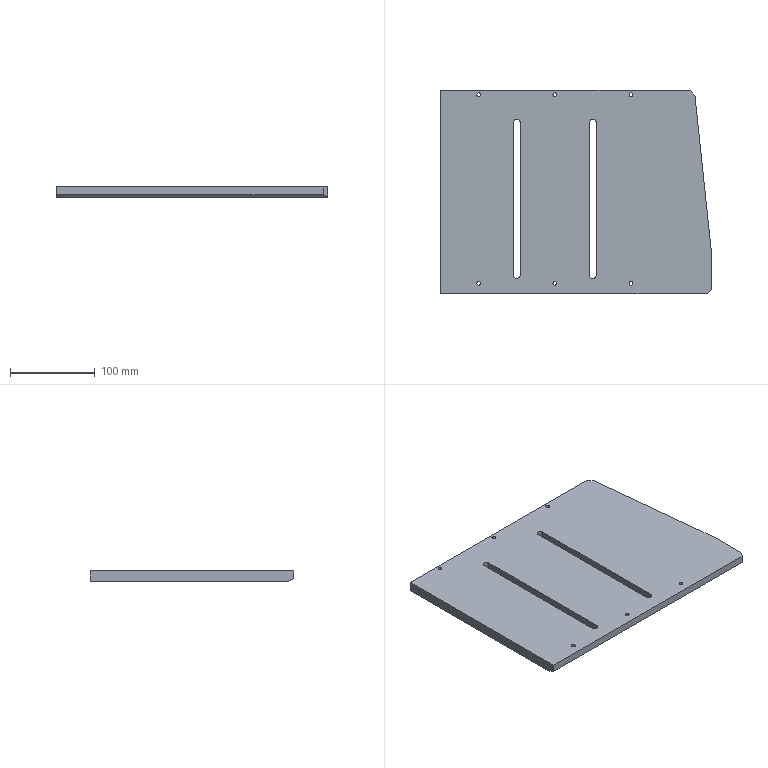Component | SolidWorks | OPW-05-007-1 | 1 solid | 42 faces | box 320 x 240 x 12 mm | volume 858405 mm3 | cylinder 16 | plane 14 | cone 12 | commonest cylinder face diameters 4.5 x12 8 x4
build123d program:
from build123d import *
from OCP.BRepFilletAPI import BRepFilletAPI_MakeChamfer

# Parameters (mm, degrees)
SKETCH1_W                                            = 320
SKETCH1_H                                            = 240
BOSS_EXTRUDE1_DEPTH                                  = 6
CUT_EXTRUDE1_REACH                                   = 202.36
COUNTERSUNK_HOLE_FOR_M4_HEX_SOCKET_COUNT_D           = 4.5
COUNTERSUNK_HOLE_FOR_M4_HEX_SOCKET_COUNT_CSINK_D     = 9.18
COUNTERSUNK_HOLE_FOR_M4_HEX_SOCKET_COUNT_CSINK_ANGLE = 90
CUT_EXTRUDE2_REACH                                   = 202.36
CHAMFER1_SIZE                                        = 6
CHAMFER1_SIZE2                                       = 3
CHAMFER2_SIZE                                        = 5
CHAMFER2_SIZE2                                       = 5.619


with BuildPart() as part:
    # Sketch1 → Boss-Extrude1 (new, symmetric)
    with BuildSketch(Plane.XY):
        Rectangle(SKETCH1_W, SKETCH1_H)
    extrude(amount=BOSS_EXTRUDE1_DEPTH, both=True)

    # Sketch2 → Cut-Extrude1 (cut, up to next)
    with BuildSketch(Plane.XY.offset(6), mode=Mode.PRIVATE) as cut_extrude1_sk1:
        with BuildLine():
            Line((-66, 82), (-66, -98))
            ThreePointArc((-66, -98), (-70, -102), (-74, -98))
            Line((-74, -98), (-74, 82))
            ThreePointArc((-74, 82), (-70, 86), (-66, 82))
        make_face()
    cut_extrude1_tool1 = extrude(cut_extrude1_sk1.sketch, amount=-CUT_EXTRUDE1_REACH, mode=Mode.PRIVATE) & part.part
    # Sketch2 → Cut-Extrude1 (cut, up to next)
    with BuildSketch(Plane.XY.offset(6), mode=Mode.PRIVATE) as cut_extrude1_sk2:
        with BuildLine():
            Line((24, 82), (24, -98))
            ThreePointArc((24, -98), (20, -102), (16, -98))
            Line((16, -98), (16, 82))
            ThreePointArc((16, 82), (20, 86), (24, 82))
        make_face()
    cut_extrude1_tool2 = extrude(cut_extrude1_sk2.sketch, amount=-CUT_EXTRUDE1_REACH, mode=Mode.PRIVATE) & part.part
    add(cut_extrude1_tool1.solids().sort_by_distance((-70, -8, 6))[0], mode=Mode.SUBTRACT)
    add(cut_extrude1_tool2.solids().sort_by_distance((20, -8, 6))[0], mode=Mode.SUBTRACT)

    # Countersunk Hole for M4 Hex Socket Count (through all)
    with Locations(Plane(origin=(0, 0, -6), x_dir=(-1, 0, 0), z_dir=(0, 0, -1))):
        with Locations((115, -108), (115, 115), (25, 115), (25, -108), (-65, 115), (-65, -108)):
            CounterSinkHole(COUNTERSUNK_HOLE_FOR_M4_HEX_SOCKET_COUNT_D / 2, COUNTERSUNK_HOLE_FOR_M4_HEX_SOCKET_COUNT_CSINK_D / 2, counter_sink_angle=COUNTERSUNK_HOLE_FOR_M4_HEX_SOCKET_COUNT_CSINK_ANGLE)

    # Sketch7 → Cut-Extrude2 (cut, up to next)
    with BuildSketch(Plane.XY.offset(6), mode=Mode.PRIVATE) as cut_extrude2_sk1:
        Polygon((140, 120), (160, -70), (160, 120), align=None)
    cut_extrude2_tool1 = extrude(cut_extrude2_sk1.sketch, amount=-CUT_EXTRUDE2_REACH, mode=Mode.PRIVATE) & part.part
    add(cut_extrude2_tool1.solids().sort_by_distance((153.333, 56.667, 6))[0], mode=Mode.SUBTRACT)

    # Chamfer1
    chamfer1_edges = [part.edges().sort_by_distance(p)[0] for p in [
        (0, -120, -6),
    ]]
    chamfer1_side = [part.faces().sort_by_distance(p)[0] for p in [
        (-2.893, -1.191, -6),
    ]]
    chamfer(chamfer1_edges, length=CHAMFER1_SIZE, length2=CHAMFER1_SIZE2, reference=chamfer1_side[0])

    # Chamfer2: one chamfer whose edges measure the first distance from different faces: ONE call of the kernel's chamfer builder (chamfer() names one face for all edges)
    chamfer2_edges_1 = [part.edges().sort_by_distance(p)[0] for p in [
        (160, -120, 1.5),
    ]]
    chamfer2_edges_2 = [part.edges().sort_by_distance(p)[0] for p in [
        (140, 120, 0),
    ]]
    chamfer2_side_2 = [part.faces().sort_by_distance(p)[0] for p in [
        (-10, 120, 0),
    ]]
    chamfer2 = BRepFilletAPI_MakeChamfer(part.part.solid().wrapped)
    for e in chamfer2_edges_1:
        chamfer2.Add(CHAMFER2_SIZE, e.wrapped)
    for e in chamfer2_edges_2:
        chamfer2.Add(CHAMFER2_SIZE, CHAMFER2_SIZE2, e.wrapped, chamfer2_side_2[0].wrapped)  # the first distance lies on this face
    add(Compound.cast(chamfer2.Shape()), mode=Mode.REPLACE)


solid = part.part

# Placed as in the assembly
solid = solid.moved(Location((-79.904, 345.999, -35), (0, 0, 0)))